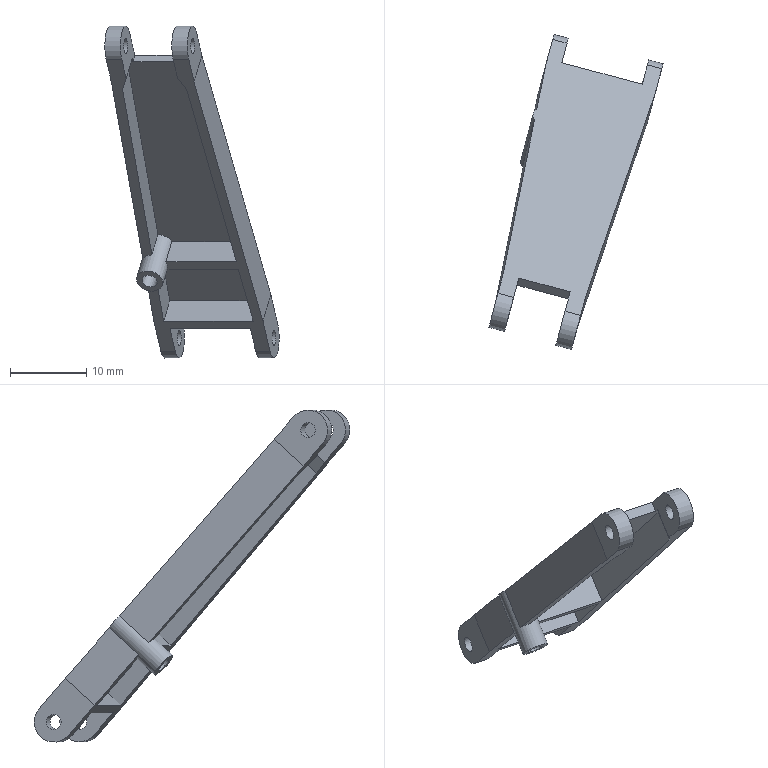Component | NX | CONNECTING_ROD | 1 solid | 40 faces | volume 1569 mm3 | plane 29 | cylinder 10 | cone 1 | commonest cylinder face diameters 2 x5 5.292 x4 3.52 x1